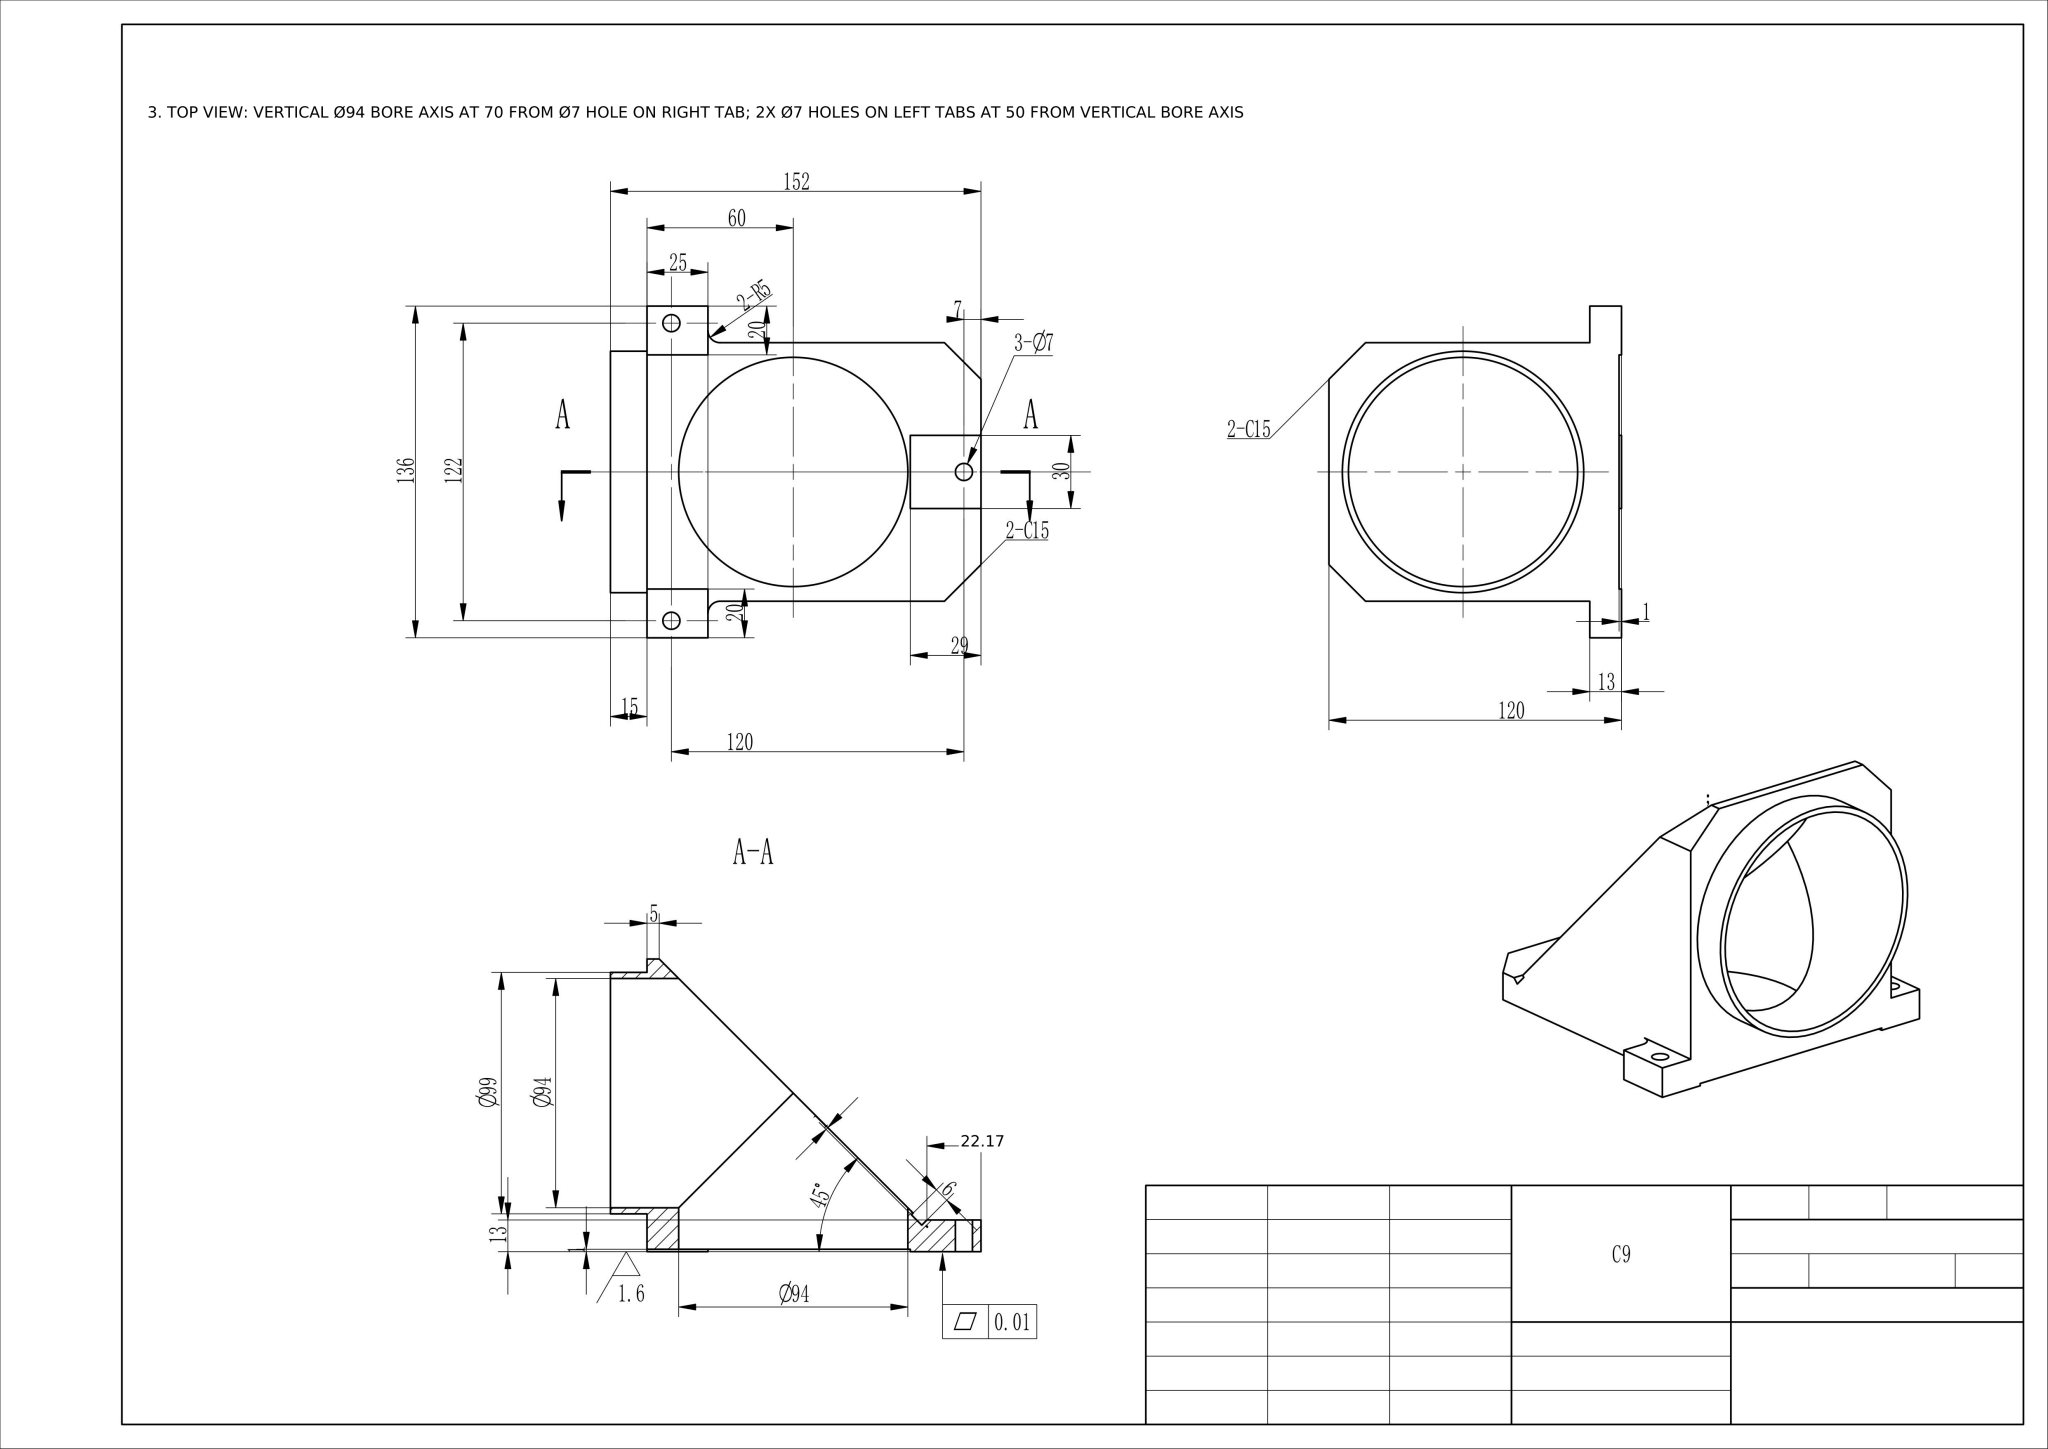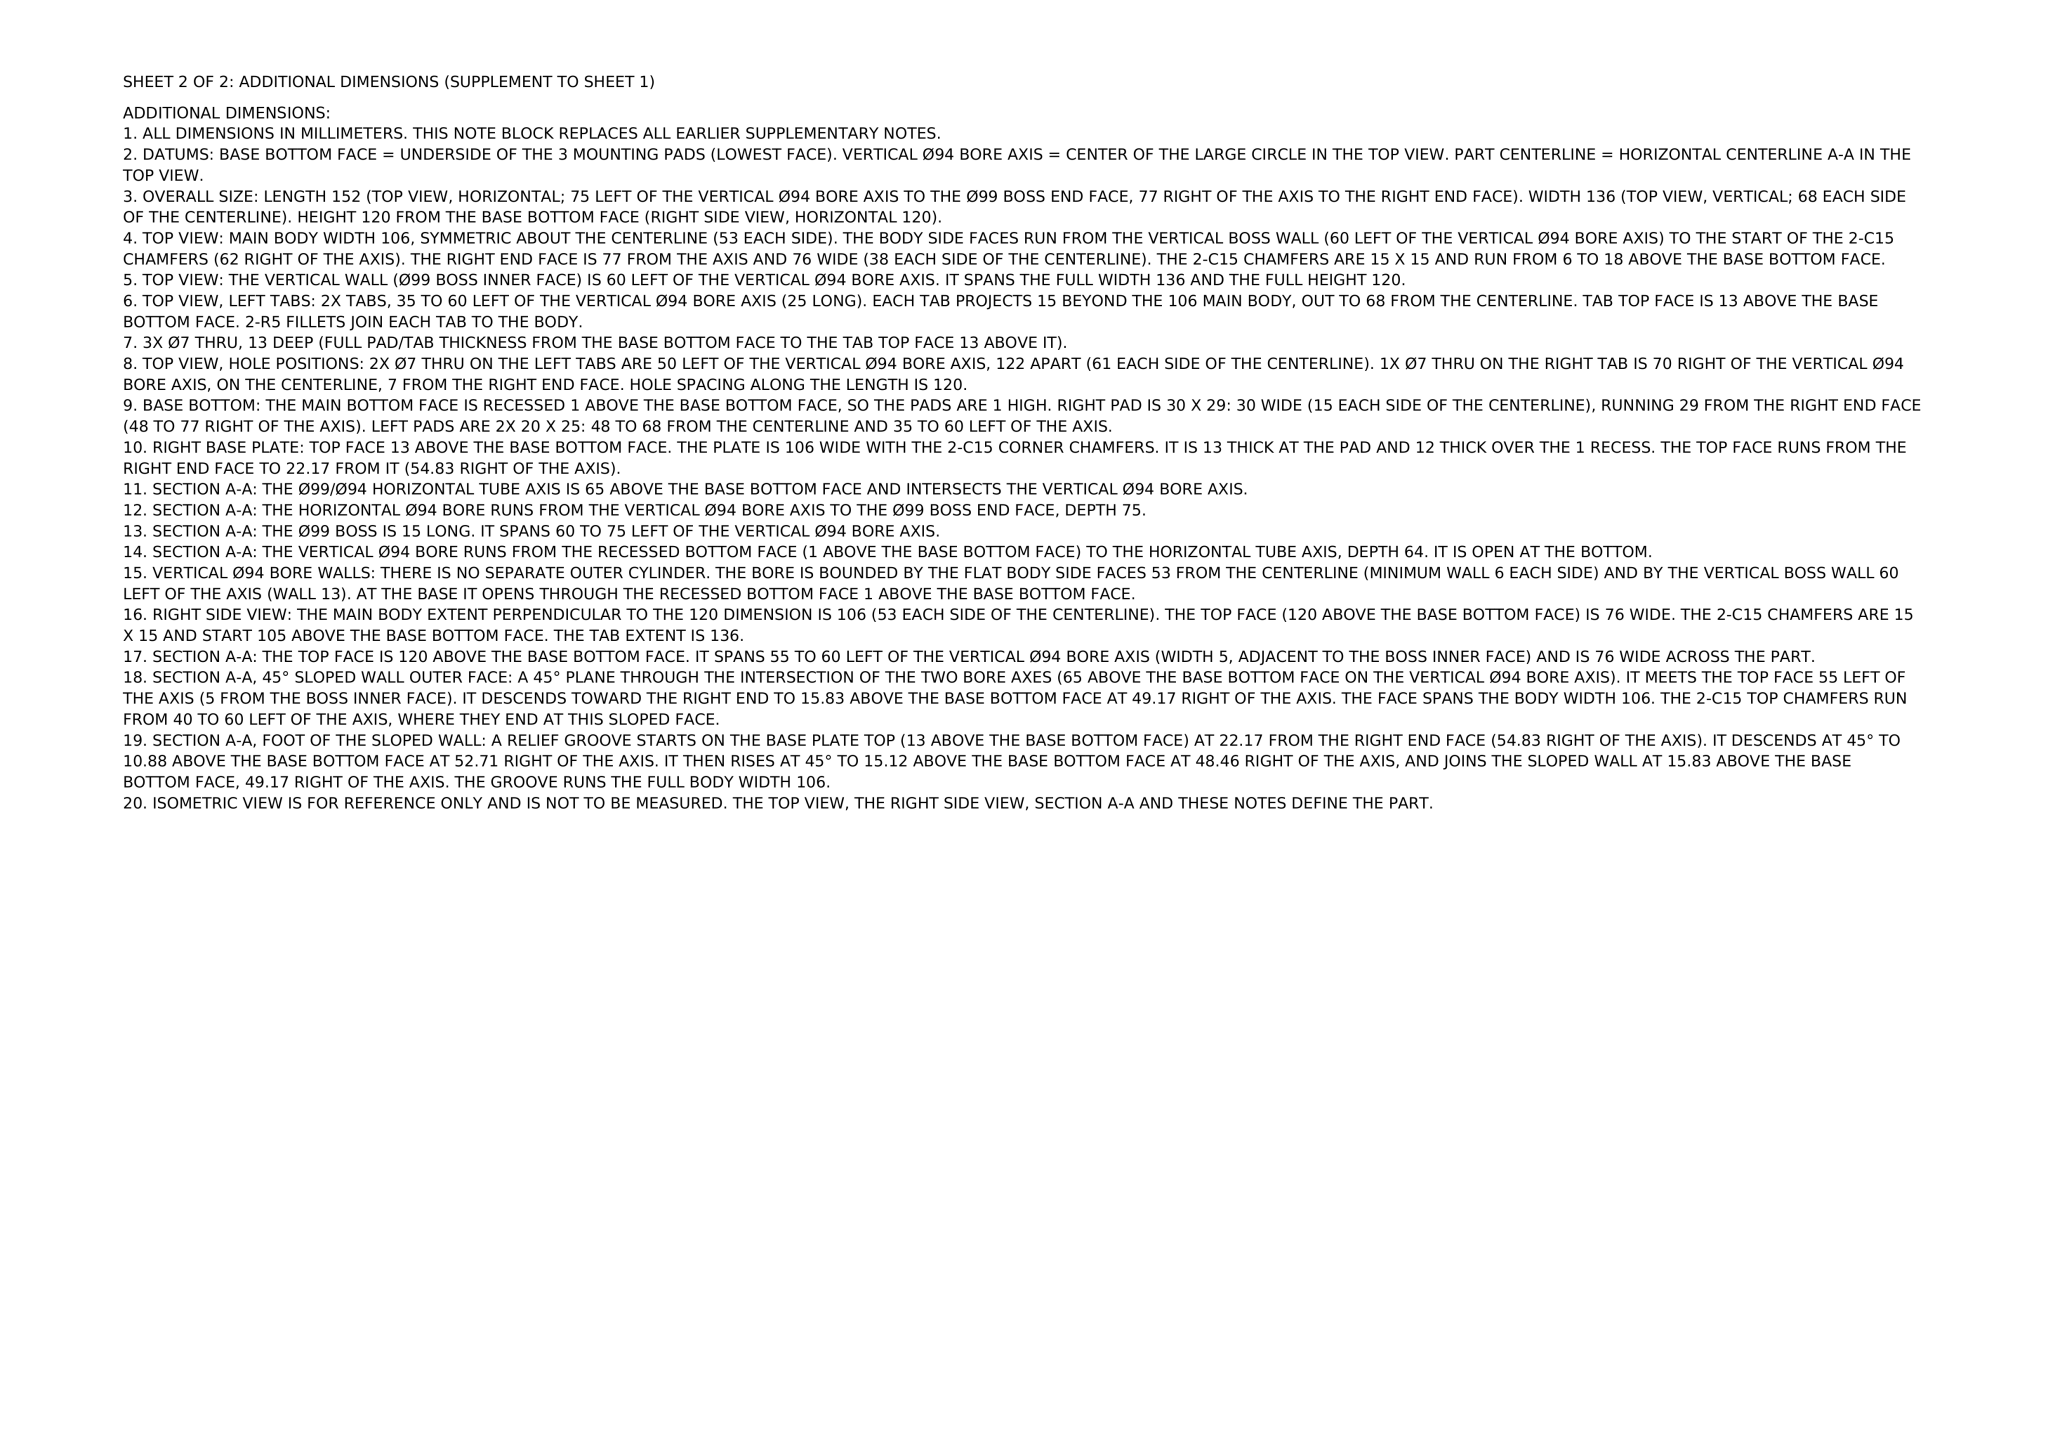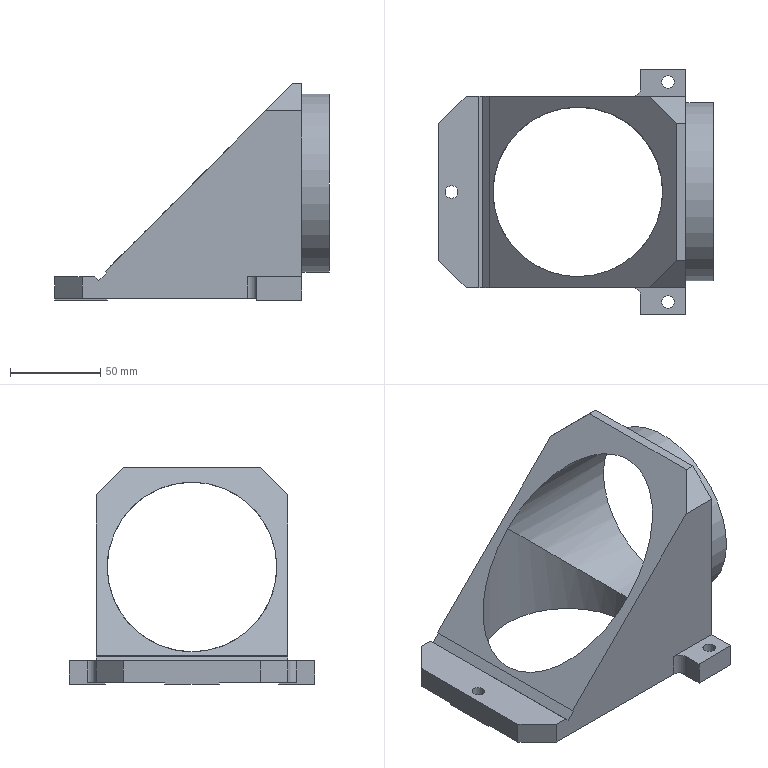Part | NX | mm | 1 solid | 41 faces | box 152 x 136 x 120 mm | volume 269167 mm3 | plane 32 | cylinder 9 | commonest cylinder face diameters 7 x3 94 x2 10 x2 99 x1 110 x1